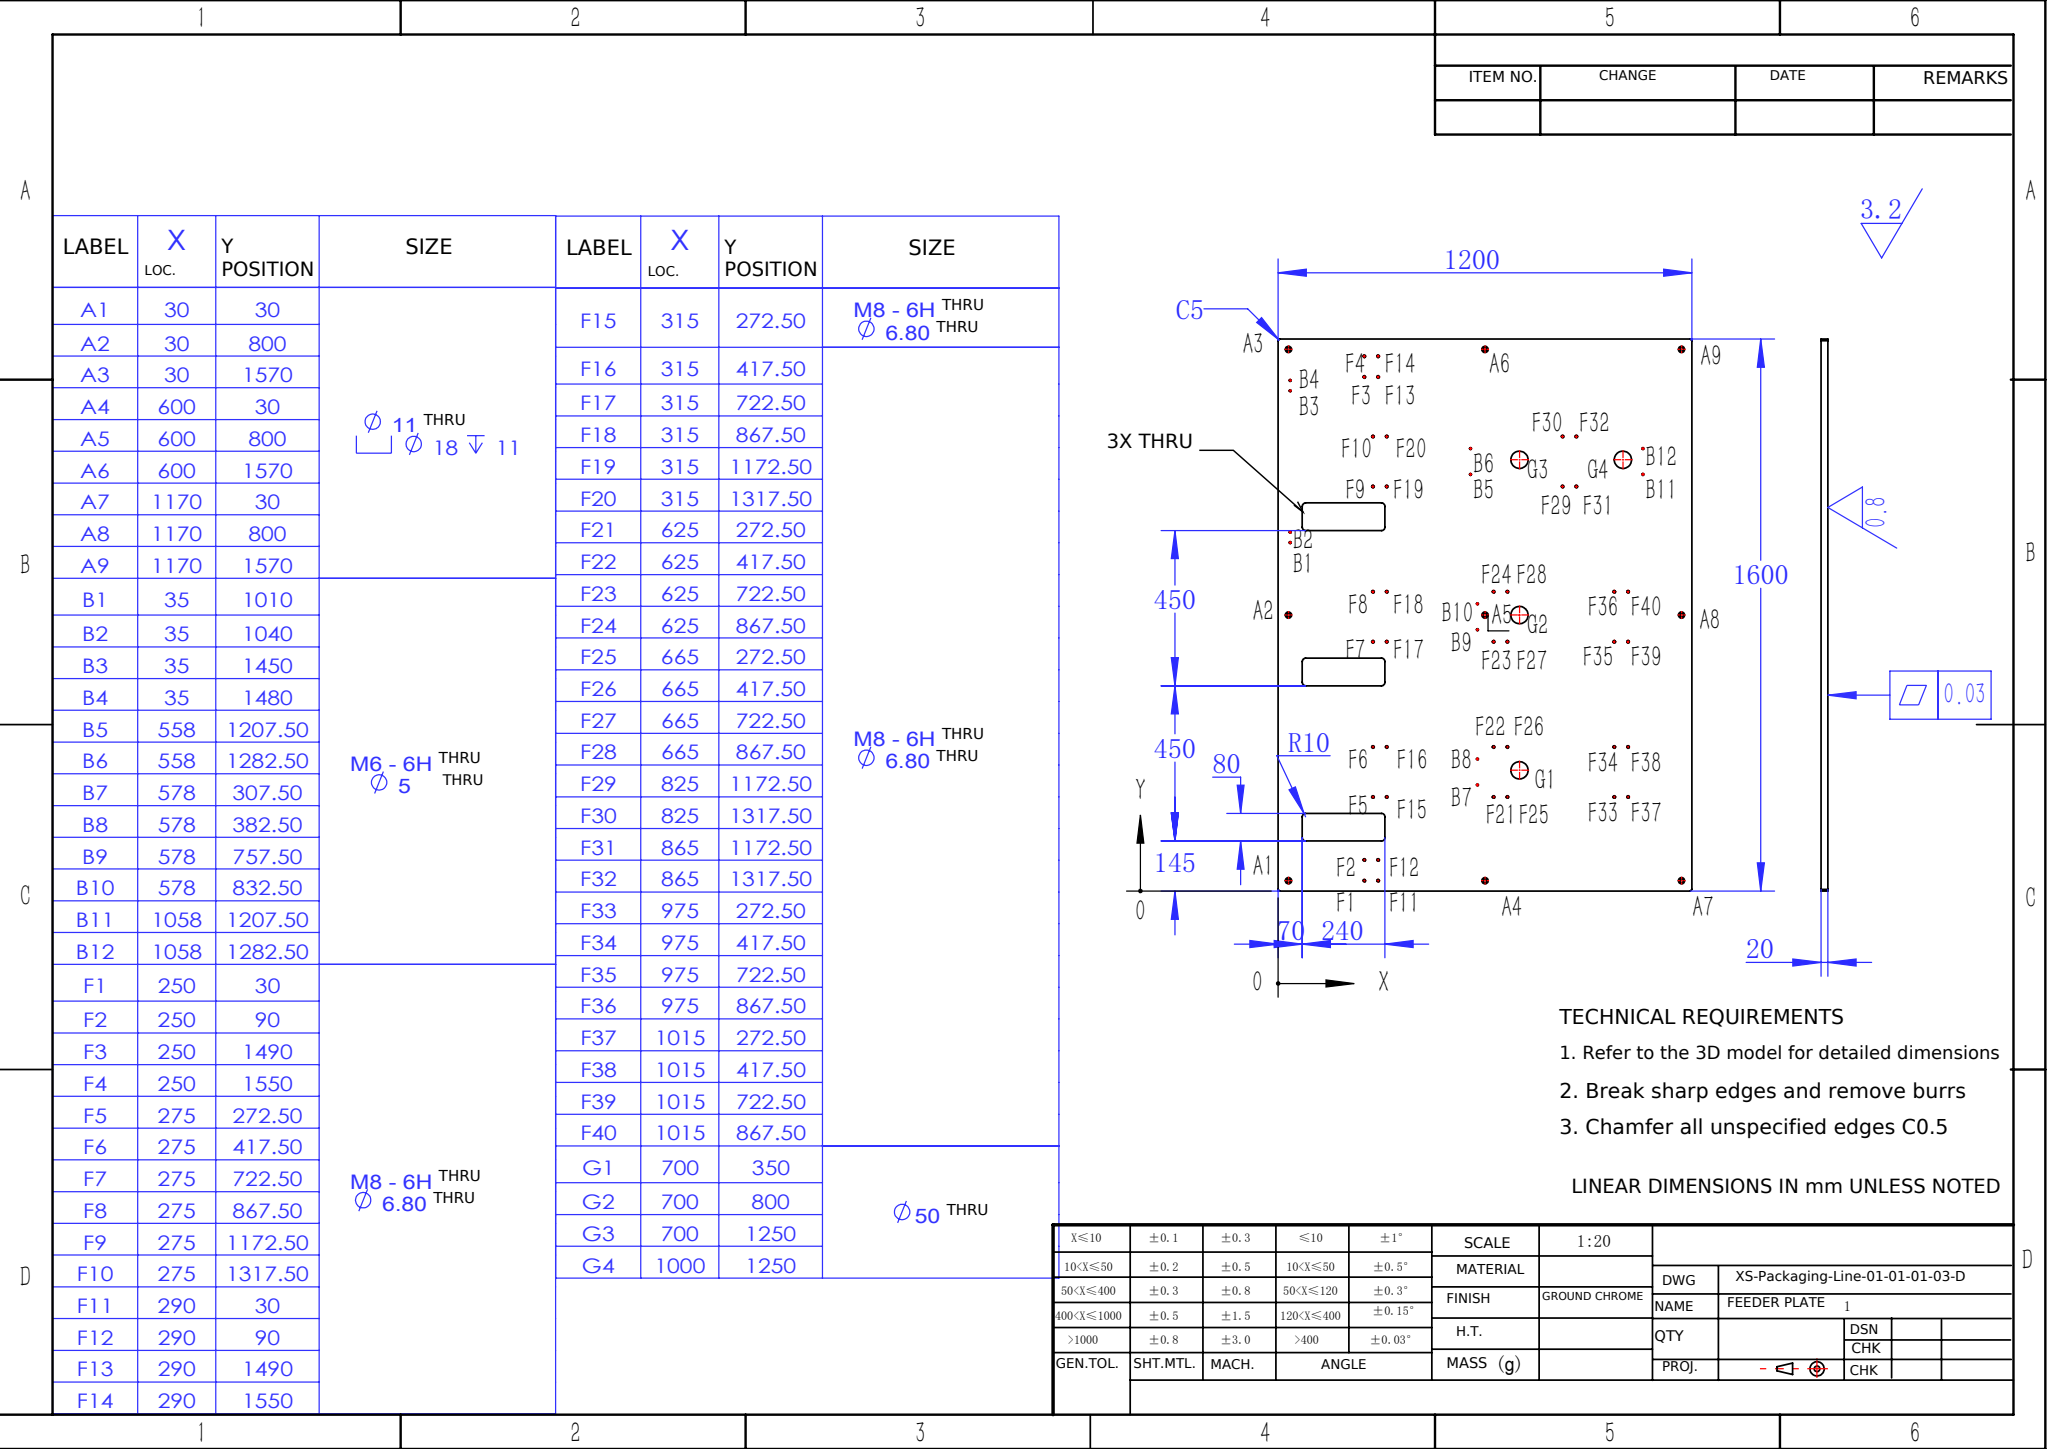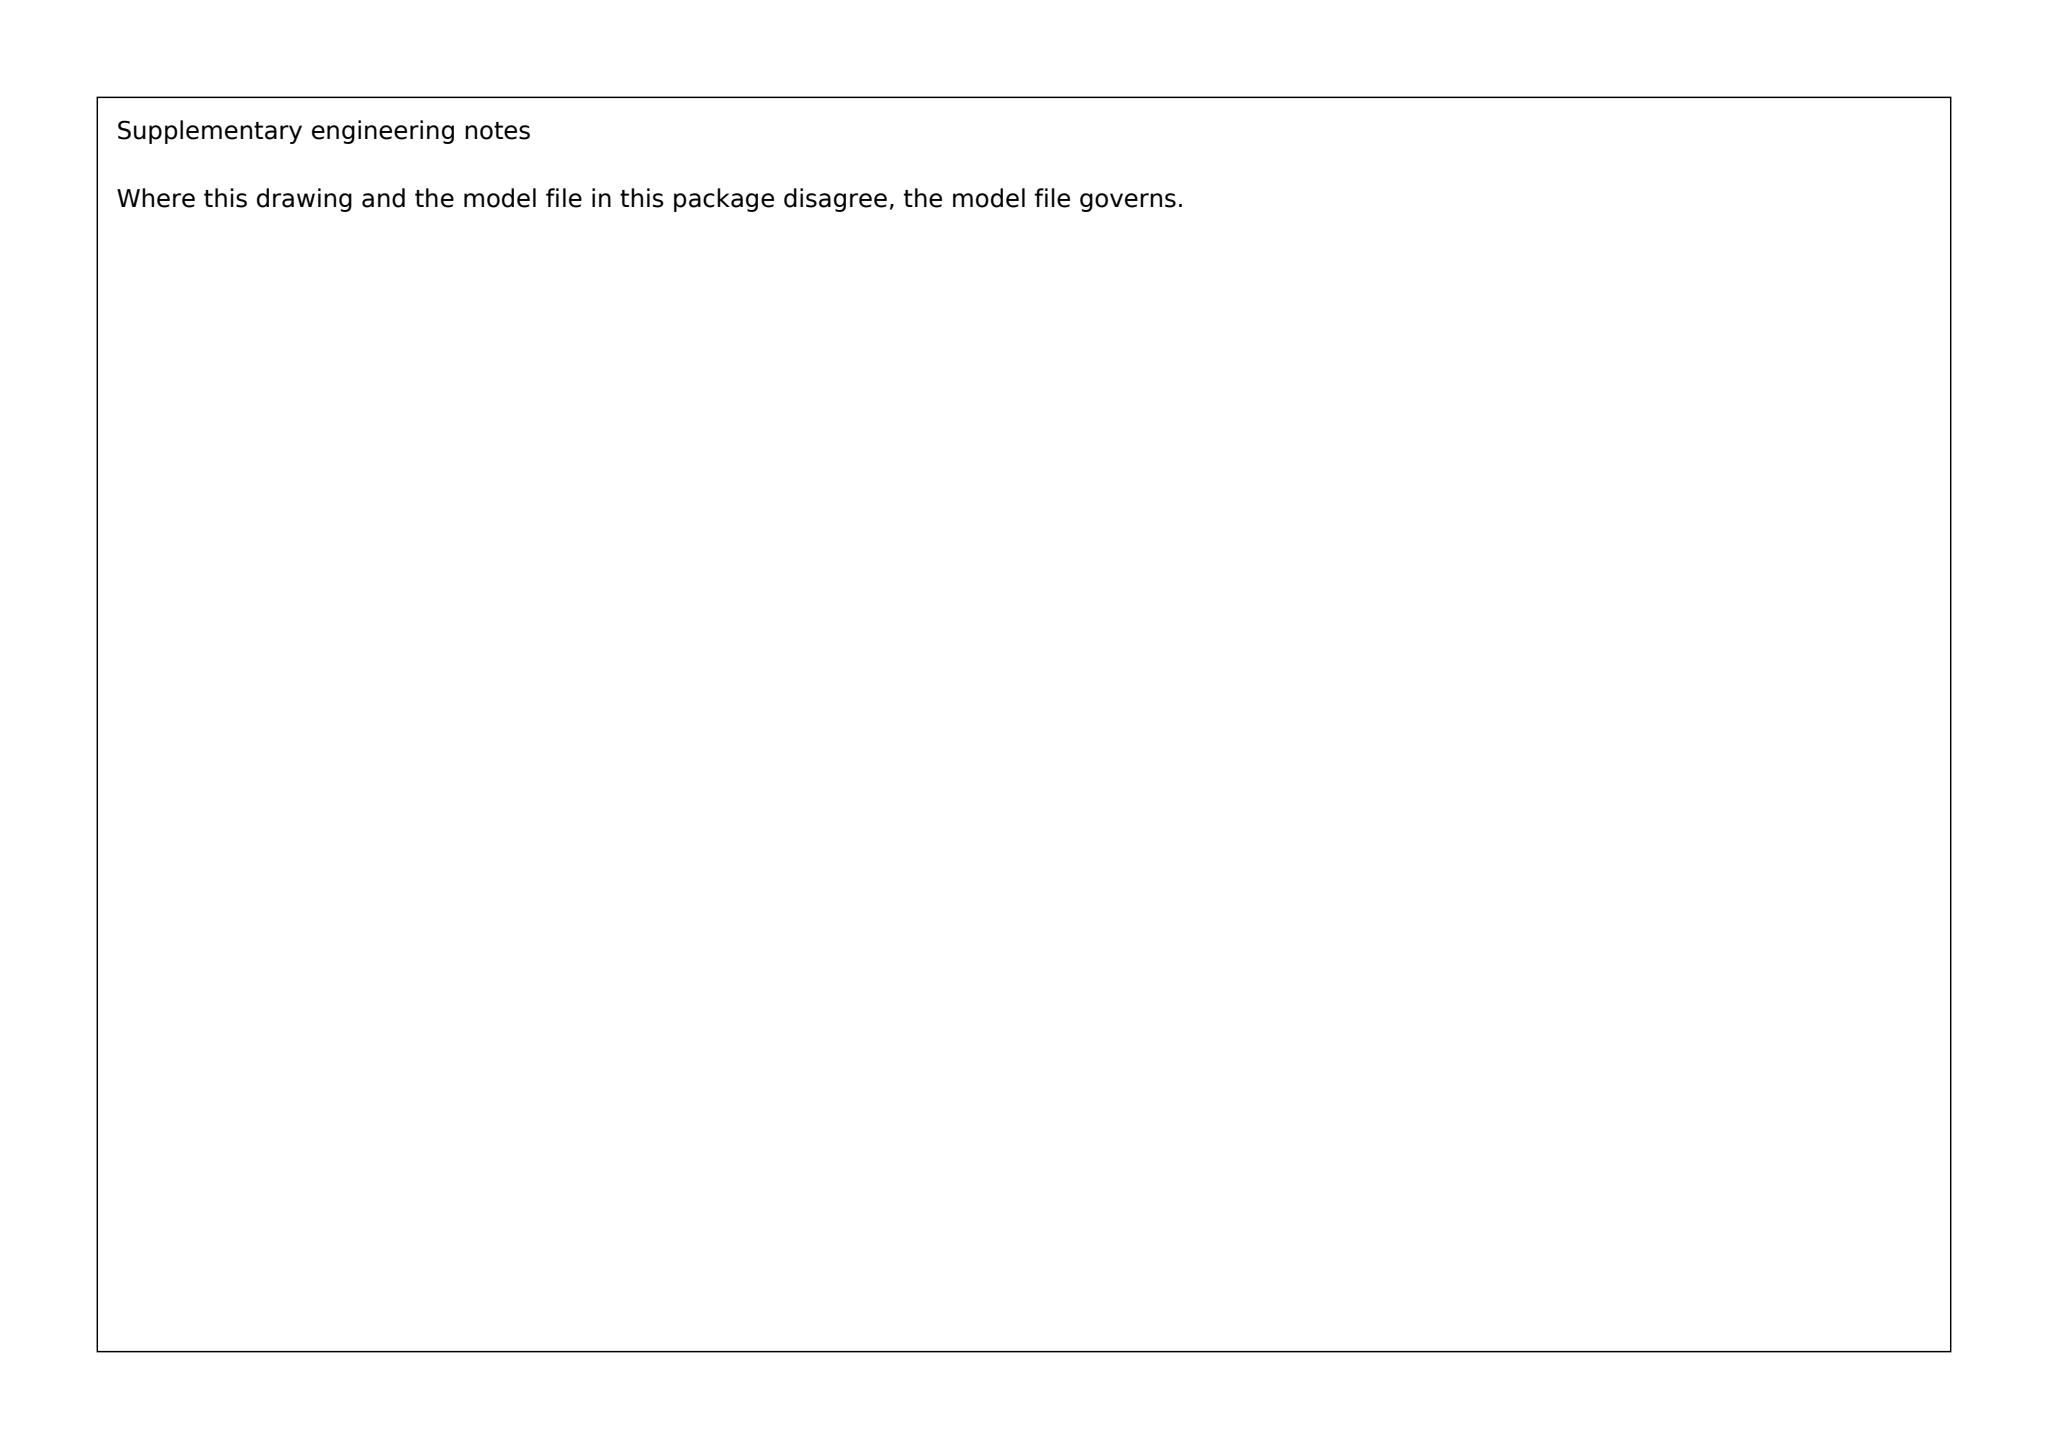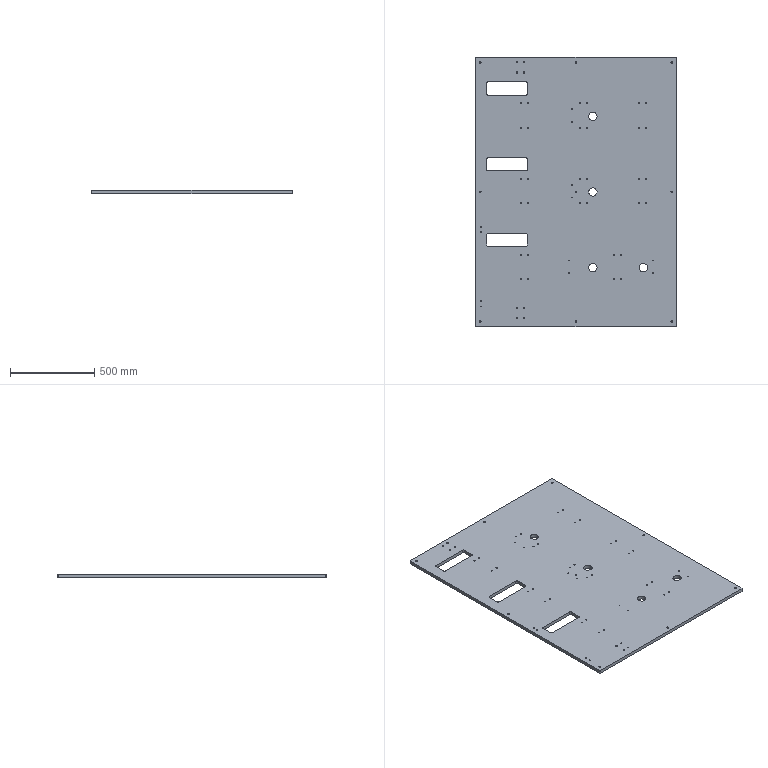Part | SolidWorks | mm | 1 solid | 191 faces | box 1200 x 1600 x 20 mm | volume 37028415 mm3 | cylinder 160 | plane 31 | commonest cylinder face diameters 6.8 x80 5 x24 18 x18 11 x18 20 x12 50 x8
build123d program:
from build123d import *

# Parameters (mm, degrees)
SKETCH1_W                                        = 2700
SKETCH1_H                                        = 1600
BOSS_EXTRUDE1_DEPTH                              = 20
SKETCH2_W                                        = 240
SKETCH2_H                                        = 80
CUT_EXTRUDE1_DEPTH                               = 1570.363
FILLET1_R                                        = 10
LPATTERN1_COUNT                                  = 3
LPATTERN1_PITCH                                  = 450
FILLET1_OF_LPATTERN1_R                           = 10
SKETCH11_W                                       = 1500
SKETCH11_H                                       = 1600
CUT_EXTRUDE2_DEPTH                               = 1570.363
CHAMFER3_SIZE                                    = 5
M10_HEX_SOCKET_HEAD_CAP_SCREW_CBORE1_D           = 11
M10_HEX_SOCKET_HEAD_CAP_SCREW_CBORE1_CBORE_D     = 18
M10_HEX_SOCKET_HEAD_CAP_SCREW_CBORE1_CBORE_DEPTH = 11
LPATTERN2_COUNT                                  = 3
LPATTERN2_PITCH                                  = 570
LPATTERN2_COUNT_DIR2                             = 3
LPATTERN2_PITCH_DIR2                             = 770
M6_TAPPED_HOLE1_D                                = 5
LPATTERN3_COUNT                                  = 2
LPATTERN3_PITCH                                  = 440
M8_TAPPED_HOLE1_D                                = 6.8
M8_TAPPED_HOLE2_D                                = 6.8
LPATTERN4_COUNT                                  = 2
LPATTERN4_PITCH                                  = 450
M6_TAPPED_HOLE2_D                                = 5
M6_TAPPED_HOLE3_D                                = 5
M8_TAPPED_HOLE3_D                                = 6.8
LPATTERN5_COUNT                                  = 2
LPATTERN5_PITCH                                  = 1460
SKETCH26_R                                       = 25
CUT_EXTRUDE3_DEPTH                               = 50
LPATTERN6_COUNT                                  = 3
LPATTERN6_PITCH                                  = 450
LPATTERN6_COUNT_DIR2                             = 2
LPATTERN6_PITCH_DIR2                             = 300


with BuildPart() as part:
    # Sketch1 → Boss-Extrude1 (new body)
    with BuildSketch(Plane.XY):
        Rectangle(SKETCH1_W, SKETCH1_H)
    extrude(amount=BOSS_EXTRUDE1_DEPTH)

    # Sketch2 → Cut-Extrude1 (cut, through all)
    with BuildSketch(Plane(origin=(0, 0, 0), x_dir=(-1, 0, 0), z_dir=(0, 0, -1))):
        with Locations((1160, 615)):
            Rectangle(SKETCH2_W, SKETCH2_H)
    cut_extrude1 = extrude(amount=-CUT_EXTRUDE1_DEPTH, mode=Mode.SUBTRACT)

    # Fillet1
    fillet1_edges = [part.edges().sort_by_distance(p)[0] for p in [
        (-1040, 575, 10),
        (-1040, 655, 10),
        (-1280, 655, 10),
        (-1280, 575, 10),
    ]]
    fillet(fillet1_edges, radius=FILLET1_R)

    # LPattern1: Cut-Extrude1 ×3
    with Locations(*[(0, -i * LPATTERN1_PITCH, 0) for i in range(1, LPATTERN1_COUNT)]):
        add(cut_extrude1, mode=Mode.SUBTRACT)

    # Fillet1 of LPattern1
    fillet1_of_lpattern1_edges = [part.edges().sort_by_distance(p)[0] for p in [
        (-1040, 125, 10),
        (-1040, 205, 10),
        (-1280, 205, 10),
        (-1280, 125, 10),
        (-1040, -325, 10),
        (-1040, -245, 10),
        (-1280, -245, 10),
        (-1280, -325, 10),
    ]]
    fillet(fillet1_of_lpattern1_edges, radius=FILLET1_OF_LPATTERN1_R)

    # Sketch11 → Cut-Extrude2 (cut, through all)
    with BuildSketch(Plane(origin=(0, 0, 0), x_dir=(-1, 0, 0), z_dir=(0, 0, -1))):
        with Locations((-600, 0)):
            Rectangle(SKETCH11_W, SKETCH11_H)
    extrude(amount=-CUT_EXTRUDE2_DEPTH, mode=Mode.SUBTRACT)

    # Chamfer3
    chamfer3_edges = [part.edges().sort_by_distance(p)[0] for p in [
        (-150, 800, 10),
        (-150, -800, 10),
        (-1350, -800, 10),
        (-1350, 800, 10),
    ]]
    chamfer(chamfer3_edges, length=CHAMFER3_SIZE)

    # M10 Hex Socket Head Cap Screw CBORE1 (through all)
    with Locations(Plane(origin=(0, 0, 0), x_dir=(-1, 0, 0), z_dir=(0, 0, -1))):
        with Locations((1320, -770)):
            m10_hex_socket_head_cap_screw_cbore1 = CounterBoreHole(M10_HEX_SOCKET_HEAD_CAP_SCREW_CBORE1_D / 2, M10_HEX_SOCKET_HEAD_CAP_SCREW_CBORE1_CBORE_D / 2, M10_HEX_SOCKET_HEAD_CAP_SCREW_CBORE1_CBORE_DEPTH)

    # LPattern2: M10 Hex Socket Head Cap Screw CBORE1 3 × 3
    with Locations(*[(i * LPATTERN2_PITCH, j * LPATTERN2_PITCH_DIR2, 0) for i in range(LPATTERN2_COUNT) for j in range(LPATTERN2_COUNT_DIR2) if (i, j) != (0, 0)]):
        add(m10_hex_socket_head_cap_screw_cbore1, mode=Mode.SUBTRACT)

    # M6 Tapped Hole1 (through all)
    with Locations(Plane(origin=(0, 0, 0), x_dir=(-1, 0, 0), z_dir=(0, 0, -1))):
        with Locations((1315, -680), (1315, -650)):
            m6_tapped_hole1 = Hole(M6_TAPPED_HOLE1_D / 2)

    # LPattern3: M6 Tapped Hole1 ×2
    with Locations(*[(0, i * LPATTERN3_PITCH, 0) for i in range(1, LPATTERN3_COUNT)]):
        add(m6_tapped_hole1, mode=Mode.SUBTRACT)

    # M8 Tapped Hole1 (through all)
    with Locations(Plane(origin=(0, 0, 0), x_dir=(-1, 0, 0), z_dir=(0, 0, -1))):
        with Locations((1035, -372.5), (1075, -372.5), (1075, -517.5), (1035, -517.5), (485, -372.5), (525, -372.5), (525, -517.5), (485, -517.5)):
            Hole(M8_TAPPED_HOLE1_D / 2)

    # M8 Tapped Hole2 (through all)
    with Locations(Plane(origin=(0, 0, 0), x_dir=(-1, 0, 0), z_dir=(0, 0, -1))):
        with Locations((335, 527.5), (375, 527.5), (685, 527.5), (725, 527.5), (1035, 527.5), (1075, 527.5), (1075, 382.5), (1035, 382.5), (725, 382.5), (685, 382.5), (375, 382.5), (335, 382.5)):
            m8_tapped_hole2 = Hole(M8_TAPPED_HOLE2_D / 2)

    # LPattern4: M8 Tapped Hole2 ×2
    with Locations(*[(0, -i * LPATTERN4_PITCH, 0) for i in range(1, LPATTERN4_COUNT)]):
        add(m8_tapped_hole2, mode=Mode.SUBTRACT)

    # M6 Tapped Hole2 (through all)
    with Locations(Plane(origin=(0, 0, 0), x_dir=(-1, 0, 0), z_dir=(0, 0, -1))):
        with Locations((292, -407.5), (292, -482.5), (792, -407.5), (792, -482.5)):
            Hole(M6_TAPPED_HOLE2_D / 2)

    # M6 Tapped Hole3 (through all)
    with Locations(Plane(origin=(0, 0, 0), x_dir=(-1, 0, 0), z_dir=(0, 0, -1))):
        with Locations((772, 42.5), (772, -32.5), (772, 492.5), (772, 417.5)):
            Hole(M6_TAPPED_HOLE3_D / 2)

    # M8 Tapped Hole3 (through all)
    with Locations(Plane(origin=(0, 0, 0), x_dir=(-1, 0, 0), z_dir=(0, 0, -1))):
        with Locations((1060, 770), (1060, 710), (1100, 770), (1100, 710)):
            m8_tapped_hole3 = Hole(M8_TAPPED_HOLE3_D / 2)

    # LPattern5: M8 Tapped Hole3 ×2
    with Locations(*[(0, -i * LPATTERN5_PITCH, 0) for i in range(1, LPATTERN5_COUNT)]):
        add(m8_tapped_hole3, mode=Mode.SUBTRACT)

    # Sketch26 → Cut-Extrude3 (cut)
    with BuildSketch(Plane(origin=(0, 0, 0), x_dir=(-1, 0, 0), z_dir=(0, 0, -1))):
        with Locations((650, 450)):
            Circle(SKETCH26_R)
    cut_extrude3 = extrude(amount=-CUT_EXTRUDE3_DEPTH, mode=Mode.SUBTRACT)

    # LPattern6: Cut-Extrude3 3 × 2, 2 skipped
    with Locations(*[(j * LPATTERN6_PITCH_DIR2, -i * LPATTERN6_PITCH, 0) for i in range(LPATTERN6_COUNT) for j in range(LPATTERN6_COUNT_DIR2) if (i, j) not in ((0, 0), (0, 1), (1, 1))]):
        add(cut_extrude3, mode=Mode.SUBTRACT)


solid = part.part